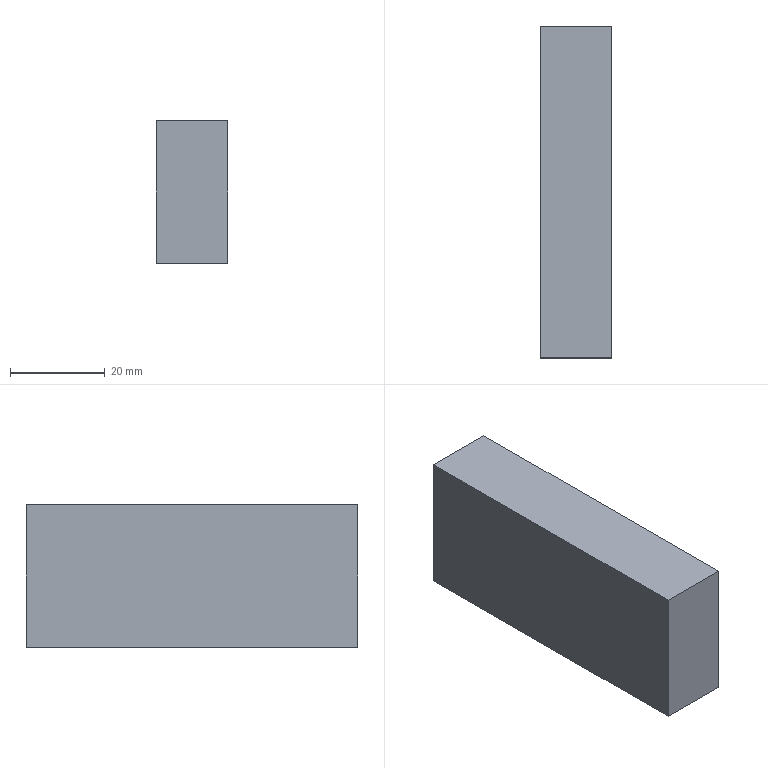Component | SolidWorks | BladeGuard-1 | 1 solid | 6 faces | box 15 x 70 x 30 mm | volume 31500 mm3 | plane 6
build123d program:
from build123d import *

# Parameters (mm, degrees)
SKETCH1_W           = 15
SKETCH1_H           = 70
BOSS_EXTRUDE1_DEPTH = 15


with BuildPart() as part:
    # Sketch1 → Boss-Extrude1 (new, symmetric)
    with BuildSketch(Plane.XY):
        Rectangle(SKETCH1_W, SKETCH1_H)
    extrude(amount=BOSS_EXTRUDE1_DEPTH, both=True)


solid = part.part

# Placed as in the assembly
solid = solid.moved(Location((-471.772, -281.766, 895.2), (0, 0, 0)))
STEP:
#1=COLOUR_RGB('',0.7922,0.8196,0.9333);
#2=FILL_AREA_STYLE_COLOUR('',#1);
#3=FILL_AREA_STYLE('',(#2));
#4=SURFACE_STYLE_FILL_AREA(#3);
#5=SURFACE_SIDE_STYLE('',(#4));
#6=SURFACE_STYLE_USAGE(.BOTH.,#5);
#7=PRESENTATION_STYLE_ASSIGNMENT((#6));
#8=CARTESIAN_POINT('',(-18.278,-12.471,34.654));
#9=VERTEX_POINT('',#8);
#10=CARTESIAN_POINT('',(-18.278,-9.715,34.654));
#11=VERTEX_POINT('',#10);
#12=CARTESIAN_POINT('',(-18.278,-12.471,34.654));
#13=DIRECTION('',(0.,1.,0.));
#14=VECTOR('',#13,39.37);
#15=LINE('',#12,#14);
#16=EDGE_CURVE('',#9,#11,#15,.T.);
#17=ORIENTED_EDGE('',*,*,#16,.T.);
#18=CARTESIAN_POINT('',(-18.278,-9.715,35.835));
#19=VERTEX_POINT('',#18);
#20=CARTESIAN_POINT('',(-18.278,-9.715,35.835));
#21=DIRECTION('',(0.,0.,-1.));
#22=VECTOR('',#21,39.37);
#23=LINE('',#20,#22);
#24=EDGE_CURVE('',#19,#11,#23,.T.);
#25=ORIENTED_EDGE('',*,*,#24,.F.);
#26=CARTESIAN_POINT('',(-18.278,-12.471,35.835));
#27=VERTEX_POINT('',#26);
#28=CARTESIAN_POINT('',(-18.278,-12.471,35.835));
#29=DIRECTION('',(0.,1.,0.));
#30=VECTOR('',#29,39.37);
#31=LINE('',#28,#30);
#32=EDGE_CURVE('',#27,#19,#31,.T.);
#33=ORIENTED_EDGE('',*,*,#32,.F.);
#34=CARTESIAN_POINT('',(-18.278,-12.471,35.835));
#35=DIRECTION('',(0.,0.,-1.));
#36=VECTOR('',#35,39.37);
#37=LINE('',#34,#36);
#38=EDGE_CURVE('',#27,#9,#37,.T.);
#39=ORIENTED_EDGE('',*,*,#38,.T.);
#40=EDGE_LOOP('',(#17,#25,#33,#39));
#41=FACE_OUTER_BOUND('',#40,.T.);
#42=CARTESIAN_POINT('',(-18.278,-12.471,35.835));
#43=DIRECTION('',(-1.,0.,-0.));
#44=DIRECTION('',(-0.,-1.,-0.));
#45=AXIS2_PLACEMENT_3D('',#42,#43,#44);
#46=PLANE('',#45);
#47=ADVANCED_FACE('',(#41),#46,.F.);
#48=CARTESIAN_POINT('',(-18.869,-9.715,34.654));
#49=VERTEX_POINT('',#48);
#50=CARTESIAN_POINT('',(-18.278,-9.715,34.654));
#51=DIRECTION('',(-1.,0.,-0.));
#52=VECTOR('',#51,39.37);
#53=LINE('',#50,#52);
#54=EDGE_CURVE('',#11,#49,#53,.T.);
#55=ORIENTED_EDGE('',*,*,#54,.T.);
#56=CARTESIAN_POINT('',(-18.869,-9.715,35.835));
#57=VERTEX_POINT('',#56);
#58=CARTESIAN_POINT('',(-18.869,-9.715,35.835));
#59=DIRECTION('',(0.,0.,-1.));
#60=VECTOR('',#59,39.37);
#61=LINE('',#58,#60);
#62=EDGE_CURVE('',#57,#49,#61,.T.);
#63=ORIENTED_EDGE('',*,*,#62,.F.);
#64=CARTESIAN_POINT('',(-18.278,-9.715,35.835));
#65=DIRECTION('',(-1.,0.,-0.));
#66=VECTOR('',#65,39.37);
#67=LINE('',#64,#66);
#68=EDGE_CURVE('',#19,#57,#67,.T.);
#69=ORIENTED_EDGE('',*,*,#68,.F.);
#70=ORIENTED_EDGE('',*,*,#24,.T.);
#71=EDGE_LOOP('',(#55,#63,#69,#70));
#72=FACE_OUTER_BOUND('',#71,.T.);
#73=CARTESIAN_POINT('',(-18.278,-9.715,35.835));
#74=DIRECTION('',(-0.,-1.,-0.));
#75=DIRECTION('',(-0.,-0.,1.));
#76=AXIS2_PLACEMENT_3D('',#73,#74,#75);
#77=PLANE('',#76);
#78=ADVANCED_FACE('',(#72),#77,.F.);
#79=CARTESIAN_POINT('',(-18.869,-12.471,34.654));
#80=VERTEX_POINT('',#79);
#81=CARTESIAN_POINT('',(-18.869,-12.471,34.654));
#82=DIRECTION('',(-0.,-1.,-0.));
#83=VECTOR('',#82,39.37);
#84=LINE('',#81,#83);
#85=EDGE_CURVE('',#49,#80,#84,.T.);
#86=ORIENTED_EDGE('',*,*,#85,.T.);
#87=CARTESIAN_POINT('',(-18.869,-12.471,35.835));
#88=VERTEX_POINT('',#87);
#89=CARTESIAN_POINT('',(-18.869,-12.471,35.835));
#90=DIRECTION('',(0.,0.,-1.));
#91=VECTOR('',#90,39.37);
#92=LINE('',#89,#91);
#93=EDGE_CURVE('',#88,#80,#92,.T.);
#94=ORIENTED_EDGE('',*,*,#93,.F.);
#95=CARTESIAN_POINT('',(-18.869,-12.471,35.835));
#96=DIRECTION('',(-0.,-1.,-0.));
#97=VECTOR('',#96,39.37);
#98=LINE('',#95,#97);
#99=EDGE_CURVE('',#57,#88,#98,.T.);
#100=ORIENTED_EDGE('',*,*,#99,.F.);
#101=ORIENTED_EDGE('',*,*,#62,.T.);
#102=EDGE_LOOP('',(#86,#94,#100,#101));
#103=FACE_OUTER_BOUND('',#102,.T.);
#104=CARTESIAN_POINT('',(-18.869,-12.471,35.835));
#105=DIRECTION('',(1.,-0.,0.));
#106=DIRECTION('',(0.,1.,0.));
#107=AXIS2_PLACEMENT_3D('',#104,#105,#106);
#108=PLANE('',#107);
#109=ADVANCED_FACE('',(#103),#108,.F.);
#110=CARTESIAN_POINT('',(-18.278,-12.471,34.654));
#111=DIRECTION('',(1.,-0.,0.));
#112=VECTOR('',#111,39.37);
#113=LINE('',#110,#112);
#114=EDGE_CURVE('',#80,#9,#113,.T.);
#115=ORIENTED_EDGE('',*,*,#114,.T.);
#116=ORIENTED_EDGE('',*,*,#38,.F.);
#117=CARTESIAN_POINT('',(-18.278,-12.471,35.835));
#118=DIRECTION('',(1.,-0.,0.));
#119=VECTOR('',#118,39.37);
#120=LINE('',#117,#119);
#121=EDGE_CURVE('',#88,#27,#120,.T.);
#122=ORIENTED_EDGE('',*,*,#121,.F.);
#123=ORIENTED_EDGE('',*,*,#93,.T.);
#124=EDGE_LOOP('',(#115,#116,#122,#123));
#125=FACE_OUTER_BOUND('',#124,.T.);
#126=CARTESIAN_POINT('',(-18.278,-12.471,35.835));
#127=DIRECTION('',(0.,1.,0.));
#128=DIRECTION('',(0.,0.,-1.));
#129=AXIS2_PLACEMENT_3D('',#126,#127,#128);
#130=PLANE('',#129);
#131=ADVANCED_FACE('',(#125),#130,.F.);
#132=ORIENTED_EDGE('',*,*,#32,.T.);
#133=ORIENTED_EDGE('',*,*,#68,.T.);
#134=ORIENTED_EDGE('',*,*,#99,.T.);
#135=ORIENTED_EDGE('',*,*,#121,.T.);
#136=EDGE_LOOP('',(#132,#133,#134,#135));
#137=FACE_OUTER_BOUND('',#136,.T.);
#138=CARTESIAN_POINT('',(-18.574,-11.093,35.835));
#139=DIRECTION('',(-0.,-0.,1.));
#140=DIRECTION('',(-1.,0.,-0.));
#141=AXIS2_PLACEMENT_3D('',#138,#139,#140);
#142=PLANE('',#141);
#143=ADVANCED_FACE('',(#137),#142,.T.);
#144=ORIENTED_EDGE('',*,*,#16,.F.);
#145=ORIENTED_EDGE('',*,*,#114,.F.);
#146=ORIENTED_EDGE('',*,*,#85,.F.);
#147=ORIENTED_EDGE('',*,*,#54,.F.);
#148=EDGE_LOOP('',(#144,#145,#146,#147));
#149=FACE_OUTER_BOUND('',#148,.T.);
#150=CARTESIAN_POINT('',(-18.574,-11.093,34.654));
#151=DIRECTION('',(-0.,-0.,1.));
#152=DIRECTION('',(-1.,0.,-0.));
#153=AXIS2_PLACEMENT_3D('',#150,#151,#152);
#154=PLANE('',#153);
#155=ADVANCED_FACE('',(#149),#154,.F.);
#156=CLOSED_SHELL('',(#47,#78,#109,#131,#143,#155));
#157=MANIFOLD_SOLID_BREP('',#156);
#158=STYLED_ITEM('',(#7),#157);
#159=(LENGTH_UNIT()NAMED_UNIT(*)SI_UNIT($,.METRE.));
#160=LENGTH_MEASURE_WITH_UNIT(LENGTH_MEASURE(0.0254),#159);
#161=DIMENSIONAL_EXPONENTS(1.,0.,0.,0.,0.,0.,0.);
#162=(CONVERSION_BASED_UNIT('',#160)LENGTH_UNIT()NAMED_UNIT(#161));
#163=UNCERTAINTY_MEASURE_WITH_UNIT(LENGTH_MEASURE(0.00001),#162,'','');
#164=(NAMED_UNIT(*)PLANE_ANGLE_UNIT()SI_UNIT($,.RADIAN.));
#165=(NAMED_UNIT(*)SI_UNIT($,.STERADIAN.)SOLID_ANGLE_UNIT());
#166=(GEOMETRIC_REPRESENTATION_CONTEXT(3)GLOBAL_UNCERTAINTY_ASSIGNED_CONTEXT((#163))GLOBAL_UNIT_ASSIGNED_CONTEXT((#162,#164,#165))REPRESENTATION_CONTEXT('',''));
#167=MECHANICAL_DESIGN_GEOMETRIC_PRESENTATION_REPRESENTATION('',(#158),#166);
#168=PRESENTATION_LAYER_ASSIGNMENT('','',(#158));
#169=CARTESIAN_POINT('',(0.,0.,0.));
#170=DIRECTION('',(0.,0.,1.));
#171=DIRECTION('',(1.,0.,0.));
#172=AXIS2_PLACEMENT_3D('',#169,#170,#171);
#173=(LENGTH_UNIT()NAMED_UNIT(*)SI_UNIT($,.METRE.));
#174=LENGTH_MEASURE_WITH_UNIT(LENGTH_MEASURE(0.0254),#173);
#175=DIMENSIONAL_EXPONENTS(1.,0.,0.,0.,0.,0.,0.);
#176=(CONVERSION_BASED_UNIT('',#174)LENGTH_UNIT()NAMED_UNIT(#175));
#177=UNCERTAINTY_MEASURE_WITH_UNIT(LENGTH_MEASURE(0.00001),#176,'','');
#178=(NAMED_UNIT(*)PLANE_ANGLE_UNIT()SI_UNIT($,.RADIAN.));
#179=(NAMED_UNIT(*)SI_UNIT($,.STERADIAN.)SOLID_ANGLE_UNIT());
#180=(GEOMETRIC_REPRESENTATION_CONTEXT(3)GLOBAL_UNCERTAINTY_ASSIGNED_CONTEXT((#177))GLOBAL_UNIT_ASSIGNED_CONTEXT((#176,#178,#179))REPRESENTATION_CONTEXT('',''));
#181=ADVANCED_BREP_SHAPE_REPRESENTATION('',(#157,#172),#180);